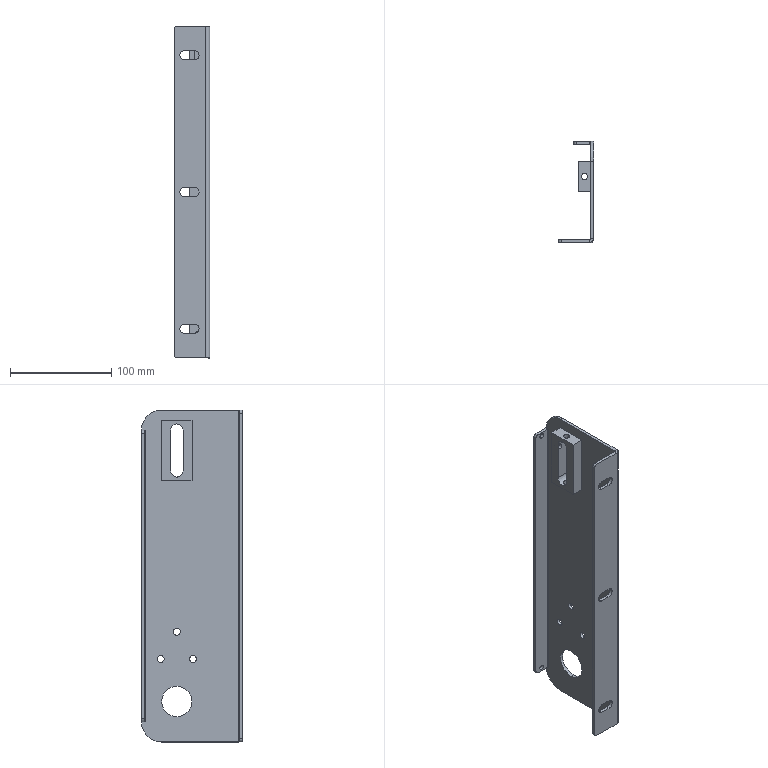Component | SolidWorks | CCD03BearingSupportPlate-1 | 1 solid | 73 faces | volume 150165 mm3 | cylinder 40 | plane 33 | commonest cylinder face diameters 9 x9 5 x6 6.8 x6 6.2 x4 6 x4 12.5 x3 30 x2 7.473 x2